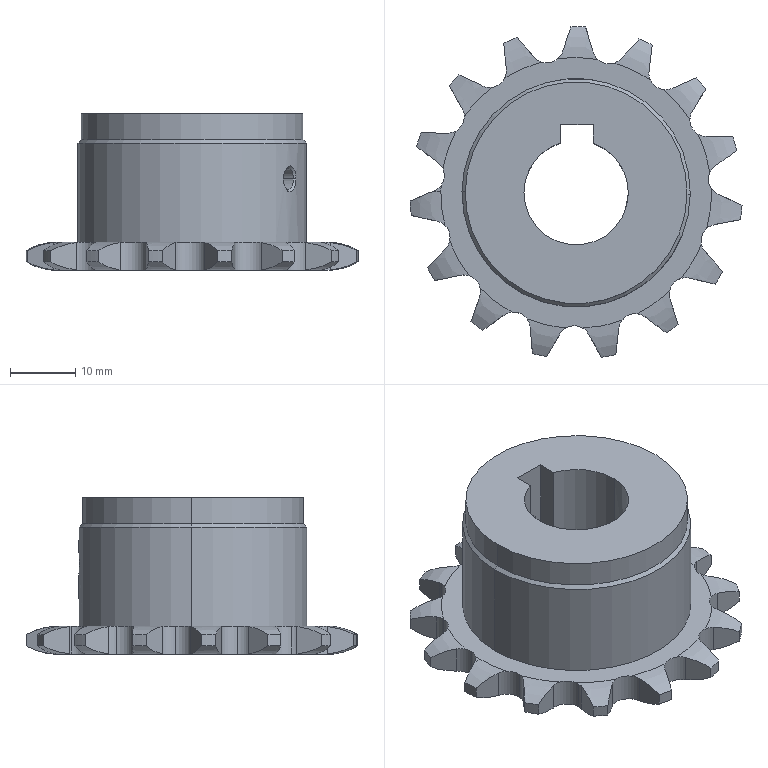Component | SolidWorks | LD101-02-35B15-d16-2 | 1 solid | 120 faces | volume 20217 mm3 | cylinder 46 | plane 36 | spline 32 | cone 6 | commonest cylinder face diameters 5.08 x20 51 x15 3.242 x4 16 x3 34 x2 35 x2